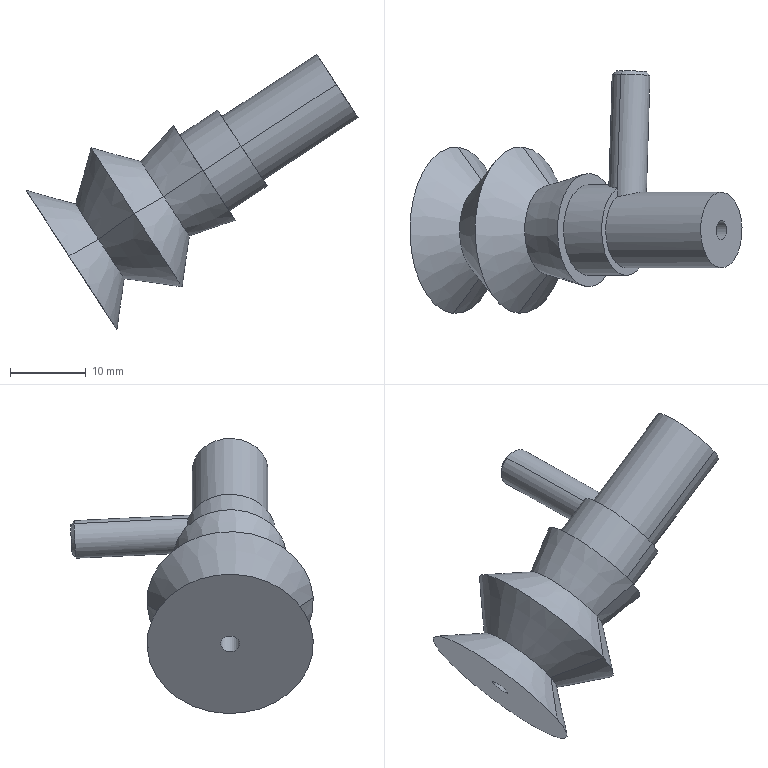Component | SolidWorks | NewSuctionCupGroup-1_SuctionCup2-1 | 1 solid | 37 faces | box 43.91 x 32.08 x 36.37 mm | volume 6180 mm3 | cylinder 19 | cone 10 | plane 8 | commonest cylinder face diameters 2.5 x7 10 x4 12 x4 5 x4
build123d program:
from build123d import *

# Parameters (mm, degrees)
SKETCH2_R               = 1.25
CUT_EXTRUDE1_DEPTH      = 61.05
CUT_EXTRUDE2_DEPTH      = 61.05
CUT_EXTRUDE2_DEPTH_BACK = 61.05
SKETCH3_W               = 23.814
SKETCH3_H               = 25.438
SKETCH4_R               = 2.5
SKETCH4_R_2             = 1.25
BOSS_EXTRUDE1_DEPTH     = 21
CHAMFER1_SIZE           = 0.5


with BuildPart() as part:
    # Sketch1 → Revolve1 (revolve)
    with BuildSketch(Plane.XY, mode=Mode.PRIVATE) as revolve1_sk:
        Polygon((0, 0), (2.5, 0), (2.5, -13), (5, -13), (5, -31), (6, -31), (6, -37), (7.489, -37), (5.895, -43.22), (11, -47.704), (5.895, -53.516), (11, -58), (0, -58), align=None)
    revolve(revolve1_sk.sketch.rotate(Axis((0, 0, 0), (0, -1, 0)), 90), axis=Axis((0, 0, 0), (0, -1, 0)))

    # Sketch2 → Cut-Extrude1 (cut, through all)
    with BuildSketch(Plane.XZ.offset(58)):
        with Locations(Location((0, 0, 0), (0, 0, 270))):
            Circle(SKETCH2_R)
    extrude(amount=-CUT_EXTRUDE1_DEPTH, mode=Mode.SUBTRACT)

    # Sketch3 → Cut-Extrude2 (cut, two sides: drawn at the far end of the back side and taken through both)
    with BuildSketch(Plane.XY.offset(-CUT_EXTRUDE2_DEPTH_BACK)):
        with Locations((1.119, -3.281)):
            Rectangle(SKETCH3_W, SKETCH3_H)
    extrude(amount=CUT_EXTRUDE2_DEPTH + CUT_EXTRUDE2_DEPTH_BACK, mode=Mode.SUBTRACT)

    # Sketch4 → Boss-Extrude1 (add)
    with BuildSketch(Plane.XY):
        with Locations((0, -31)):
            Circle(SKETCH4_R)
        with Locations((0, -31)):
            Circle(SKETCH4_R_2, mode=Mode.SUBTRACT)
    extrude(amount=BOSS_EXTRUDE1_DEPTH)

    # Chamfer1
    chamfer1_edges = [part.edges().sort_by_distance(p)[0] for p in [
        (-2.5, -31, 21),
    ]]
    chamfer(chamfer1_edges, length=CHAMFER1_SIZE)


solid = part.part

# Placed as in the assembly
solid = solid.moved(Location((-65.517, 19.546, -13.641), (-92.654, 1.733, -123.125)))